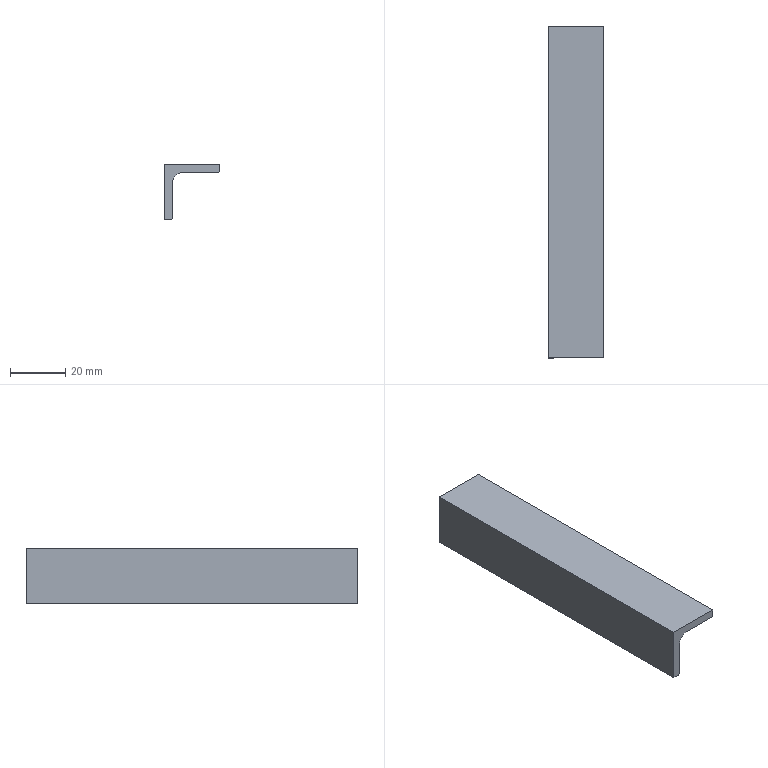Component | SolidWorks | THK-A1026AngleSteel20x20x120-4 | 1 solid | 11 faces | box 20 x 120 x 20 mm | volume 13584 mm3 | plane 8 | cylinder 3 | commonest cylinder face diameters 2 x2 7 x1 | material Q235A
build123d program:
from build123d import *

# Parameters (mm, degrees)
EXTRUDE_THIN1_DEPTH = 60
FILLET1_R           = 3.5
FILLET2_R           = 1


with BuildPart() as part:
    # Sketch1 → Extrude-Thin1 (new, symmetric)
    with BuildSketch(Plane(origin=(0, 0, 0), x_dir=(1, 0, 0), z_dir=(0, 1, 0))):
        Polygon((0, 20), (0, 0), (20, 0), (20, 3), (3, 3), (3, 20), align=None)
    extrude(amount=EXTRUDE_THIN1_DEPTH, both=True)

    # Fillet1
    fillet1_edges = [part.edges().sort_by_distance(p)[0] for p in [
        (3, 0, -3),
    ]]
    fillet(fillet1_edges, radius=FILLET1_R)

    # Fillet2
    fillet2_edges = [part.edges().sort_by_distance(p)[0] for p in [
        (3, 0, -20),
        (20, 0, -3),
    ]]
    fillet(fillet2_edges, radius=FILLET2_R)


solid = part.part

# Placed as in the assembly
solid = solid.moved(Location((-130, -101, -371), (0, 0, 0)))
STEP:
#1=COLOUR_RGB('',0.7922,0.8196,0.9333);
#2=FILL_AREA_STYLE_COLOUR('',#1);
#3=FILL_AREA_STYLE('',(#2));
#4=SURFACE_STYLE_FILL_AREA(#3);
#5=SURFACE_SIDE_STYLE('',(#4));
#6=SURFACE_STYLE_USAGE(.BOTH.,#5);
#7=PRESENTATION_STYLE_ASSIGNMENT((#6));
#8=CARTESIAN_POINT('',(-5.118,-6.339,-14.606));
#9=VERTEX_POINT('',#8);
#10=CARTESIAN_POINT('',(-4.331,-6.339,-14.606));
#11=VERTEX_POINT('',#10);
#12=CARTESIAN_POINT('',(-5.118,-6.339,-14.606));
#13=DIRECTION('',(1.,0.,0.));
#14=VECTOR('',#13,39.37);
#15=LINE('',#12,#14);
#16=EDGE_CURVE('',#9,#11,#15,.T.);
#17=ORIENTED_EDGE('',*,*,#16,.T.);
#18=CARTESIAN_POINT('',(-4.331,-1.614,-14.606));
#19=VERTEX_POINT('',#18);
#20=CARTESIAN_POINT('',(-4.331,-1.614,-14.606));
#21=DIRECTION('',(0.,-1.,0.));
#22=VECTOR('',#21,39.37);
#23=LINE('',#20,#22);
#24=EDGE_CURVE('',#19,#11,#23,.T.);
#25=ORIENTED_EDGE('',*,*,#24,.F.);
#26=CARTESIAN_POINT('',(-5.118,-1.614,-14.606));
#27=VERTEX_POINT('',#26);
#28=CARTESIAN_POINT('',(-5.118,-1.614,-14.606));
#29=DIRECTION('',(1.,0.,0.));
#30=VECTOR('',#29,39.37);
#31=LINE('',#28,#30);
#32=EDGE_CURVE('',#27,#19,#31,.T.);
#33=ORIENTED_EDGE('',*,*,#32,.F.);
#34=CARTESIAN_POINT('',(-5.118,-1.614,-14.606));
#35=DIRECTION('',(0.,-1.,0.));
#36=VECTOR('',#35,39.37);
#37=LINE('',#34,#36);
#38=EDGE_CURVE('',#27,#9,#37,.T.);
#39=ORIENTED_EDGE('',*,*,#38,.T.);
#40=EDGE_LOOP('',(#17,#25,#33,#39));
#41=FACE_OUTER_BOUND('',#40,.T.);
#42=CARTESIAN_POINT('',(-5.118,-1.614,-14.606));
#43=DIRECTION('',(0.,0.,-1.));
#44=DIRECTION('',(-1.,0.,0.));
#45=AXIS2_PLACEMENT_3D('',#42,#43,#44);
#46=PLANE('',#45);
#47=ADVANCED_FACE('',(#41),#46,.F.);
#48=CARTESIAN_POINT('',(-4.331,-6.339,-14.685));
#49=VERTEX_POINT('',#48);
#50=CARTESIAN_POINT('',(-4.331,-6.339,-14.724));
#51=DIRECTION('',(0.,0.,1.));
#52=VECTOR('',#51,39.37);
#53=LINE('',#50,#52);
#54=EDGE_CURVE('',#49,#11,#53,.T.);
#55=ORIENTED_EDGE('',*,*,#54,.F.);
#56=CARTESIAN_POINT('',(-4.331,-1.614,-14.685));
#57=VERTEX_POINT('',#56);
#58=CARTESIAN_POINT('',(-4.331,-1.614,-14.685));
#59=DIRECTION('',(0.,1.,0.));
#60=VECTOR('',#59,39.37);
#61=LINE('',#58,#60);
#62=EDGE_CURVE('',#49,#57,#61,.T.);
#63=ORIENTED_EDGE('',*,*,#62,.T.);
#64=CARTESIAN_POINT('',(-4.331,-1.614,-14.724));
#65=DIRECTION('',(0.,0.,1.));
#66=VECTOR('',#65,39.37);
#67=LINE('',#64,#66);
#68=EDGE_CURVE('',#57,#19,#67,.T.);
#69=ORIENTED_EDGE('',*,*,#68,.T.);
#70=ORIENTED_EDGE('',*,*,#24,.T.);
#71=EDGE_LOOP('',(#55,#63,#69,#70));
#72=FACE_OUTER_BOUND('',#71,.T.);
#73=CARTESIAN_POINT('',(-4.331,-1.614,-14.724));
#74=DIRECTION('',(1.,0.,0.));
#75=DIRECTION('',(0.,0.,-1.));
#76=AXIS2_PLACEMENT_3D('',#73,#74,#75);
#77=PLANE('',#76);
#78=ADVANCED_FACE('',(#72),#77,.T.);
#79=CARTESIAN_POINT('',(-4.862,-1.614,-14.724));
#80=VERTEX_POINT('',#79);
#81=CARTESIAN_POINT('',(-4.37,-1.614,-14.724));
#82=VERTEX_POINT('',#81);
#83=CARTESIAN_POINT('',(-5.118,-1.614,-14.724));
#84=DIRECTION('',(1.,0.,0.));
#85=VECTOR('',#84,39.37);
#86=LINE('',#83,#85);
#87=EDGE_CURVE('',#80,#82,#86,.T.);
#88=ORIENTED_EDGE('',*,*,#87,.T.);
#89=CARTESIAN_POINT('',(-4.37,-6.339,-14.724));
#90=VERTEX_POINT('',#89);
#91=CARTESIAN_POINT('',(-4.37,-1.614,-14.724));
#92=DIRECTION('',(0.,-1.,0.));
#93=VECTOR('',#92,39.37);
#94=LINE('',#91,#93);
#95=EDGE_CURVE('',#82,#90,#94,.T.);
#96=ORIENTED_EDGE('',*,*,#95,.T.);
#97=CARTESIAN_POINT('',(-4.862,-6.339,-14.724));
#98=VERTEX_POINT('',#97);
#99=CARTESIAN_POINT('',(-5.118,-6.339,-14.724));
#100=DIRECTION('',(1.,0.,0.));
#101=VECTOR('',#100,39.37);
#102=LINE('',#99,#101);
#103=EDGE_CURVE('',#98,#90,#102,.T.);
#104=ORIENTED_EDGE('',*,*,#103,.F.);
#105=CARTESIAN_POINT('',(-4.862,-1.614,-14.724));
#106=DIRECTION('',(0.,1.,0.));
#107=VECTOR('',#106,39.37);
#108=LINE('',#105,#107);
#109=EDGE_CURVE('',#98,#80,#108,.T.);
#110=ORIENTED_EDGE('',*,*,#109,.T.);
#111=EDGE_LOOP('',(#88,#96,#104,#110));
#112=FACE_OUTER_BOUND('',#111,.T.);
#113=CARTESIAN_POINT('',(-5.118,-1.614,-14.724));
#114=DIRECTION('',(0.,0.,-1.));
#115=DIRECTION('',(-1.,0.,0.));
#116=AXIS2_PLACEMENT_3D('',#113,#114,#115);
#117=PLANE('',#116);
#118=ADVANCED_FACE('',(#112),#117,.T.);
#119=CARTESIAN_POINT('',(-5.,-6.339,-15.354));
#120=VERTEX_POINT('',#119);
#121=CARTESIAN_POINT('',(-5.,-6.339,-14.862));
#122=VERTEX_POINT('',#121);
#123=CARTESIAN_POINT('',(-5.,-6.339,-15.394));
#124=DIRECTION('',(-0.,0.,1.));
#125=VECTOR('',#124,39.37);
#126=LINE('',#123,#125);
#127=EDGE_CURVE('',#120,#122,#126,.T.);
#128=ORIENTED_EDGE('',*,*,#127,.F.);
#129=CARTESIAN_POINT('',(-5.,-1.614,-15.354));
#130=VERTEX_POINT('',#129);
#131=CARTESIAN_POINT('',(-5.,-1.614,-15.354));
#132=DIRECTION('',(0.,1.,0.));
#133=VECTOR('',#132,39.37);
#134=LINE('',#131,#133);
#135=EDGE_CURVE('',#120,#130,#134,.T.);
#136=ORIENTED_EDGE('',*,*,#135,.T.);
#137=CARTESIAN_POINT('',(-5.,-1.614,-14.862));
#138=VERTEX_POINT('',#137);
#139=CARTESIAN_POINT('',(-5.,-1.614,-15.394));
#140=DIRECTION('',(-0.,0.,1.));
#141=VECTOR('',#140,39.37);
#142=LINE('',#139,#141);
#143=EDGE_CURVE('',#130,#138,#142,.T.);
#144=ORIENTED_EDGE('',*,*,#143,.T.);
#145=CARTESIAN_POINT('',(-5.,-6.339,-14.862));
#146=DIRECTION('',(0.,-1.,0.));
#147=VECTOR('',#146,39.37);
#148=LINE('',#145,#147);
#149=EDGE_CURVE('',#138,#122,#148,.T.);
#150=ORIENTED_EDGE('',*,*,#149,.T.);
#151=EDGE_LOOP('',(#128,#136,#144,#150));
#152=FACE_OUTER_BOUND('',#151,.T.);
#153=CARTESIAN_POINT('',(-5.,-1.614,-15.394));
#154=DIRECTION('',(1.,0.,0.));
#155=DIRECTION('',(0.,0.,-1.));
#156=AXIS2_PLACEMENT_3D('',#153,#154,#155);
#157=PLANE('',#156);
#158=ADVANCED_FACE('',(#152),#157,.T.);
#159=CARTESIAN_POINT('',(-5.118,-1.614,-15.394));
#160=VERTEX_POINT('',#159);
#161=CARTESIAN_POINT('',(-5.039,-1.614,-15.394));
#162=VERTEX_POINT('',#161);
#163=CARTESIAN_POINT('',(-5.118,-1.614,-15.394));
#164=DIRECTION('',(1.,0.,0.));
#165=VECTOR('',#164,39.37);
#166=LINE('',#163,#165);
#167=EDGE_CURVE('',#160,#162,#166,.T.);
#168=ORIENTED_EDGE('',*,*,#167,.T.);
#169=CARTESIAN_POINT('',(-5.039,-6.339,-15.394));
#170=VERTEX_POINT('',#169);
#171=CARTESIAN_POINT('',(-5.039,-1.614,-15.394));
#172=DIRECTION('',(0.,-1.,0.));
#173=VECTOR('',#172,39.37);
#174=LINE('',#171,#173);
#175=EDGE_CURVE('',#162,#170,#174,.T.);
#176=ORIENTED_EDGE('',*,*,#175,.T.);
#177=CARTESIAN_POINT('',(-5.118,-6.339,-15.394));
#178=VERTEX_POINT('',#177);
#179=CARTESIAN_POINT('',(-5.118,-6.339,-15.394));
#180=DIRECTION('',(1.,0.,0.));
#181=VECTOR('',#180,39.37);
#182=LINE('',#179,#181);
#183=EDGE_CURVE('',#178,#170,#182,.T.);
#184=ORIENTED_EDGE('',*,*,#183,.F.);
#185=CARTESIAN_POINT('',(-5.118,-1.614,-15.394));
#186=DIRECTION('',(0.,-1.,0.));
#187=VECTOR('',#186,39.37);
#188=LINE('',#185,#187);
#189=EDGE_CURVE('',#160,#178,#188,.T.);
#190=ORIENTED_EDGE('',*,*,#189,.F.);
#191=EDGE_LOOP('',(#168,#176,#184,#190));
#192=FACE_OUTER_BOUND('',#191,.T.);
#193=CARTESIAN_POINT('',(-5.118,-1.614,-15.394));
#194=DIRECTION('',(0.,0.,-1.));
#195=DIRECTION('',(-1.,0.,0.));
#196=AXIS2_PLACEMENT_3D('',#193,#194,#195);
#197=PLANE('',#196);
#198=ADVANCED_FACE('',(#192),#197,.T.);
#199=CARTESIAN_POINT('',(-5.118,-6.339,-15.394));
#200=DIRECTION('',(-0.,0.,1.));
#201=VECTOR('',#200,39.37);
#202=LINE('',#199,#201);
#203=EDGE_CURVE('',#178,#9,#202,.T.);
#204=ORIENTED_EDGE('',*,*,#203,.T.);
#205=ORIENTED_EDGE('',*,*,#38,.F.);
#206=CARTESIAN_POINT('',(-5.118,-1.614,-15.394));
#207=DIRECTION('',(-0.,0.,1.));
#208=VECTOR('',#207,39.37);
#209=LINE('',#206,#208);
#210=EDGE_CURVE('',#160,#27,#209,.T.);
#211=ORIENTED_EDGE('',*,*,#210,.F.);
#212=ORIENTED_EDGE('',*,*,#189,.T.);
#213=EDGE_LOOP('',(#204,#205,#211,#212));
#214=FACE_OUTER_BOUND('',#213,.T.);
#215=CARTESIAN_POINT('',(-5.118,-1.614,-15.394));
#216=DIRECTION('',(1.,0.,0.));
#217=DIRECTION('',(0.,0.,-1.));
#218=AXIS2_PLACEMENT_3D('',#215,#216,#217);
#219=PLANE('',#218);
#220=ADVANCED_FACE('',(#214),#219,.F.);
#221=ORIENTED_EDGE('',*,*,#143,.F.);
#222=CARTESIAN_POINT('',(-5.039,-1.614,-15.354));
#223=DIRECTION('',(0.,1.,0.));
#224=DIRECTION('',(0.,0.,-1.));
#225=AXIS2_PLACEMENT_3D('',#222,#223,#224);
#226=CIRCLE('',#225,0.03937);
#227=EDGE_CURVE('',#130,#162,#226,.T.);
#228=ORIENTED_EDGE('',*,*,#227,.T.);
#229=ORIENTED_EDGE('',*,*,#167,.F.);
#230=ORIENTED_EDGE('',*,*,#210,.T.);
#231=ORIENTED_EDGE('',*,*,#32,.T.);
#232=ORIENTED_EDGE('',*,*,#68,.F.);
#233=CARTESIAN_POINT('',(-4.37,-1.614,-14.685));
#234=DIRECTION('',(0.,1.,0.));
#235=DIRECTION('',(0.,0.,-1.));
#236=AXIS2_PLACEMENT_3D('',#233,#234,#235);
#237=CIRCLE('',#236,0.03937);
#238=EDGE_CURVE('',#57,#82,#237,.T.);
#239=ORIENTED_EDGE('',*,*,#238,.T.);
#240=ORIENTED_EDGE('',*,*,#87,.F.);
#241=CARTESIAN_POINT('',(-4.862,-1.614,-14.862));
#242=DIRECTION('',(0.,-1.,0.));
#243=DIRECTION('',(0.,0.,-1.));
#244=AXIS2_PLACEMENT_3D('',#241,#242,#243);
#245=CIRCLE('',#244,0.1378);
#246=EDGE_CURVE('',#80,#138,#245,.T.);
#247=ORIENTED_EDGE('',*,*,#246,.T.);
#248=EDGE_LOOP('',(#221,#228,#229,#230,#231,#232,#239,#240,#247));
#249=FACE_OUTER_BOUND('',#248,.T.);
#250=CARTESIAN_POINT('',(-5.118,-1.614,-14.606));
#251=DIRECTION('',(0.,-1.,0.));
#252=DIRECTION('',(-1.,0.,0.));
#253=AXIS2_PLACEMENT_3D('',#250,#251,#252);
#254=PLANE('',#253);
#255=ADVANCED_FACE('',(#249),#254,.F.);
#256=ORIENTED_EDGE('',*,*,#183,.T.);
#257=CARTESIAN_POINT('',(-5.039,-6.339,-15.354));
#258=DIRECTION('',(0.,-1.,0.));
#259=DIRECTION('',(0.,0.,-1.));
#260=AXIS2_PLACEMENT_3D('',#257,#258,#259);
#261=CIRCLE('',#260,0.03937);
#262=EDGE_CURVE('',#170,#120,#261,.T.);
#263=ORIENTED_EDGE('',*,*,#262,.T.);
#264=ORIENTED_EDGE('',*,*,#127,.T.);
#265=CARTESIAN_POINT('',(-4.862,-6.339,-14.862));
#266=DIRECTION('',(0.,1.,0.));
#267=DIRECTION('',(0.,0.,-1.));
#268=AXIS2_PLACEMENT_3D('',#265,#266,#267);
#269=CIRCLE('',#268,0.1378);
#270=EDGE_CURVE('',#122,#98,#269,.T.);
#271=ORIENTED_EDGE('',*,*,#270,.T.);
#272=ORIENTED_EDGE('',*,*,#103,.T.);
#273=CARTESIAN_POINT('',(-4.37,-6.339,-14.685));
#274=DIRECTION('',(0.,-1.,0.));
#275=DIRECTION('',(0.,0.,-1.));
#276=AXIS2_PLACEMENT_3D('',#273,#274,#275);
#277=CIRCLE('',#276,0.03937);
#278=EDGE_CURVE('',#90,#49,#277,.T.);
#279=ORIENTED_EDGE('',*,*,#278,.T.);
#280=ORIENTED_EDGE('',*,*,#54,.T.);
#281=ORIENTED_EDGE('',*,*,#16,.F.);
#282=ORIENTED_EDGE('',*,*,#203,.F.);
#283=EDGE_LOOP('',(#256,#263,#264,#271,#272,#279,#280,#281,#282));
#284=FACE_OUTER_BOUND('',#283,.T.);
#285=CARTESIAN_POINT('',(-5.118,-6.339,-14.606));
#286=DIRECTION('',(0.,-1.,0.));
#287=DIRECTION('',(-1.,0.,0.));
#288=AXIS2_PLACEMENT_3D('',#285,#286,#287);
#289=PLANE('',#288);
#290=ADVANCED_FACE('',(#284),#289,.T.);
#291=ORIENTED_EDGE('',*,*,#246,.F.);
#292=ORIENTED_EDGE('',*,*,#109,.F.);
#293=ORIENTED_EDGE('',*,*,#270,.F.);
#294=ORIENTED_EDGE('',*,*,#149,.F.);
#295=EDGE_LOOP('',(#291,#292,#293,#294));
#296=FACE_OUTER_BOUND('',#295,.T.);
#297=CARTESIAN_POINT('',(-4.862,-1.614,-14.862));
#298=DIRECTION('',(0.,1.,0.));
#299=DIRECTION('',(0.,0.,1.));
#300=AXIS2_PLACEMENT_3D('',#297,#298,#299);
#301=CYLINDRICAL_SURFACE('',#300,0.1378);
#302=ADVANCED_FACE('',(#296),#301,.F.);
#303=ORIENTED_EDGE('',*,*,#227,.F.);
#304=ORIENTED_EDGE('',*,*,#135,.F.);
#305=ORIENTED_EDGE('',*,*,#262,.F.);
#306=ORIENTED_EDGE('',*,*,#175,.F.);
#307=EDGE_LOOP('',(#303,#304,#305,#306));
#308=FACE_OUTER_BOUND('',#307,.T.);
#309=CARTESIAN_POINT('',(-5.039,-1.614,-15.354));
#310=DIRECTION('',(0.,-1.,0.));
#311=DIRECTION('',(0.,0.,-1.));
#312=AXIS2_PLACEMENT_3D('',#309,#310,#311);
#313=CYLINDRICAL_SURFACE('',#312,0.03937);
#314=ADVANCED_FACE('',(#308),#313,.T.);
#315=ORIENTED_EDGE('',*,*,#238,.F.);
#316=ORIENTED_EDGE('',*,*,#62,.F.);
#317=ORIENTED_EDGE('',*,*,#278,.F.);
#318=ORIENTED_EDGE('',*,*,#95,.F.);
#319=EDGE_LOOP('',(#315,#316,#317,#318));
#320=FACE_OUTER_BOUND('',#319,.T.);
#321=CARTESIAN_POINT('',(-4.37,-1.614,-14.685));
#322=DIRECTION('',(0.,-1.,0.));
#323=DIRECTION('',(0.,0.,-1.));
#324=AXIS2_PLACEMENT_3D('',#321,#322,#323);
#325=CYLINDRICAL_SURFACE('',#324,0.03937);
#326=ADVANCED_FACE('',(#320),#325,.T.);
#327=CLOSED_SHELL('',(#47,#78,#118,#158,#198,#220,#255,#290,#302,#314,#326));
#328=MANIFOLD_SOLID_BREP('',#327);
#329=STYLED_ITEM('',(#7),#328);
#330=(LENGTH_UNIT()NAMED_UNIT(*)SI_UNIT($,.METRE.));
#331=LENGTH_MEASURE_WITH_UNIT(LENGTH_MEASURE(0.0254),#330);
#332=DIMENSIONAL_EXPONENTS(1.,0.,0.,0.,0.,0.,0.);
#333=(CONVERSION_BASED_UNIT('',#331)LENGTH_UNIT()NAMED_UNIT(#332));
#334=UNCERTAINTY_MEASURE_WITH_UNIT(LENGTH_MEASURE(0.00001),#333,'','');
#335=(NAMED_UNIT(*)PLANE_ANGLE_UNIT()SI_UNIT($,.RADIAN.));
#336=(NAMED_UNIT(*)SI_UNIT($,.STERADIAN.)SOLID_ANGLE_UNIT());
#337=(GEOMETRIC_REPRESENTATION_CONTEXT(3)GLOBAL_UNCERTAINTY_ASSIGNED_CONTEXT((#334))GLOBAL_UNIT_ASSIGNED_CONTEXT((#333,#335,#336))REPRESENTATION_CONTEXT('',''));
#338=MECHANICAL_DESIGN_GEOMETRIC_PRESENTATION_REPRESENTATION('',(#329),#337);
#339=CARTESIAN_POINT('',(0.,0.,0.));
#340=DIRECTION('',(0.,0.,1.));
#341=DIRECTION('',(1.,0.,0.));
#342=AXIS2_PLACEMENT_3D('',#339,#340,#341);
#343=(LENGTH_UNIT()NAMED_UNIT(*)SI_UNIT($,.METRE.));
#344=LENGTH_MEASURE_WITH_UNIT(LENGTH_MEASURE(0.0254),#343);
#345=DIMENSIONAL_EXPONENTS(1.,0.,0.,0.,0.,0.,0.);
#346=(CONVERSION_BASED_UNIT('',#344)LENGTH_UNIT()NAMED_UNIT(#345));
#347=UNCERTAINTY_MEASURE_WITH_UNIT(LENGTH_MEASURE(0.00001),#346,'','');
#348=(NAMED_UNIT(*)PLANE_ANGLE_UNIT()SI_UNIT($,.RADIAN.));
#349=(NAMED_UNIT(*)SI_UNIT($,.STERADIAN.)SOLID_ANGLE_UNIT());
#350=(GEOMETRIC_REPRESENTATION_CONTEXT(3)GLOBAL_UNCERTAINTY_ASSIGNED_CONTEXT((#347))GLOBAL_UNIT_ASSIGNED_CONTEXT((#346,#348,#349))REPRESENTATION_CONTEXT('',''));
#351=ADVANCED_BREP_SHAPE_REPRESENTATION('',(#328,#342),#350);
#352=PRESENTATION_LAYER_ASSIGNMENT('','',(#329));